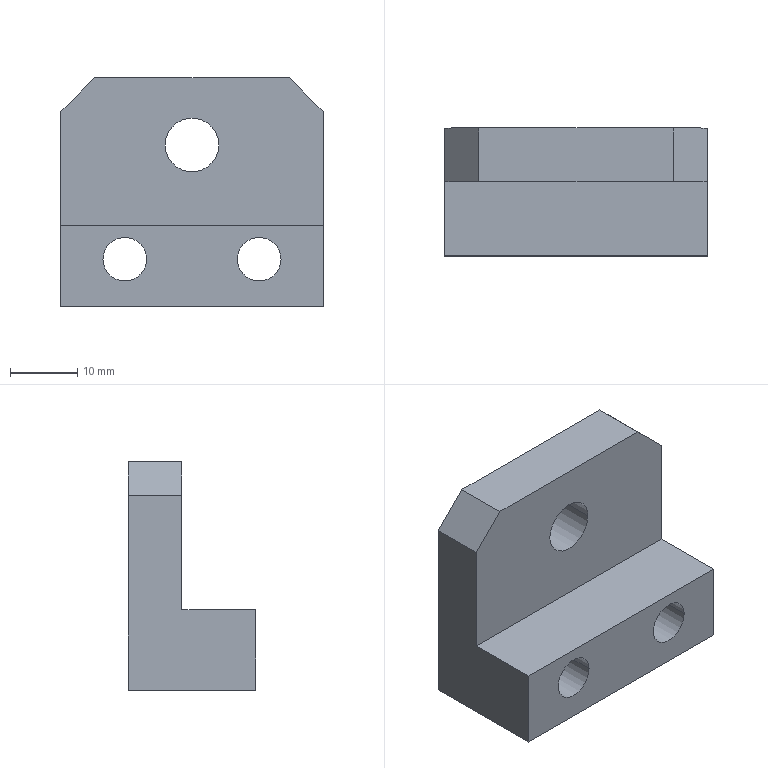Component | SolidWorks | AdjustmentBlock-1 | 1 solid | 22 faces | box 39 x 19 x 34 mm | volume 13089 mm3 | plane 12 | cylinder 10 | commonest cylinder face diameters 11 x4 6.5 x4 8 x2
build123d program:
from build123d import *

# Parameters (mm, degrees)
SKETCH1_W                                          = 39
SKETCH1_H                                          = 34
BOSS_EXTRUDE1_DEPTH                                = 19
SKETCH2_W                                          = 39
SKETCH2_H                                          = 22
CUT_EXTRUDE1_DEPTH                                 = 11
HOLE_SIZE_ACCORDING_TO_TYPE_1_OF_HEXAG_D           = 6.5
HOLE_SIZE_ACCORDING_TO_TYPE_1_OF_HEXAG_CBORE_D     = 11
HOLE_SIZE_ACCORDING_TO_TYPE_1_OF_HEXAG_CBORE_DEPTH = 6.5
SKETCH5_R                                          = 4
CUT_EXTRUDE2_DEPTH                                 = 11
CHAMFER1_SIZE                                      = 5


with BuildPart() as part:
    # Sketch1 → Boss-Extrude1 (new body)
    with BuildSketch(Plane.XY):
        Rectangle(SKETCH1_W, SKETCH1_H)
    extrude(amount=BOSS_EXTRUDE1_DEPTH)

    # Sketch2 → Cut-Extrude1 (cut)
    with BuildSketch(Plane(origin=(0, 0, 0), x_dir=(-1, 0, 0), z_dir=(0, 0, -1))):
        with Locations((0, 6)):
            Rectangle(SKETCH2_W, SKETCH2_H)
    extrude(amount=-CUT_EXTRUDE1_DEPTH, mode=Mode.SUBTRACT)

    # Hole Size _according to_ Type 1 of Hexag (through all)
    with Locations(Plane(origin=(-10, -10, 19), x_dir=(1, 0, 0), z_dir=(0, 0, 1))):
        with Locations((0, 0), (20, 0)):
            CounterBoreHole(HOLE_SIZE_ACCORDING_TO_TYPE_1_OF_HEXAG_D / 2, HOLE_SIZE_ACCORDING_TO_TYPE_1_OF_HEXAG_CBORE_D / 2, HOLE_SIZE_ACCORDING_TO_TYPE_1_OF_HEXAG_CBORE_DEPTH)

    # Sketch5 → Cut-Extrude2 (cut)
    with BuildSketch(Plane.XY.offset(19)):
        with Locations((0, 7)):
            Circle(SKETCH5_R)
    extrude(amount=-CUT_EXTRUDE2_DEPTH, mode=Mode.SUBTRACT)

    # Chamfer1
    chamfer1_edges = [part.edges().sort_by_distance(p)[0] for p in [
        (-19.5, 17, 15),
        (19.5, 17, 15),
    ]]
    chamfer(chamfer1_edges, length=CHAMFER1_SIZE)


solid = part.part

# Placed as in the assembly
solid = solid.moved(Location((-48.047, 25.96, 8), (-90, 0, 180)))
STEP:
#1=COLOUR_RGB('',0.7922,0.8196,0.9333);
#2=FILL_AREA_STYLE_COLOUR('',#1);
#3=FILL_AREA_STYLE('',(#2));
#4=SURFACE_STYLE_FILL_AREA(#3);
#5=SURFACE_SIDE_STYLE('',(#4));
#6=SURFACE_STYLE_USAGE(.BOTH.,#5);
#7=PRESENTATION_STYLE_ASSIGNMENT((#6));
#8=CARTESIAN_POINT('',(-2.049,1.455,0.5906));
#9=VERTEX_POINT('',#8);
#10=CARTESIAN_POINT('',(-1.734,1.455,0.5906));
#11=VERTEX_POINT('',#10);
#12=CARTESIAN_POINT('',(-1.892,1.455,0.5906));
#13=DIRECTION('',(0.,-1.,0.));
#14=DIRECTION('',(1.,0.,0.));
#15=AXIS2_PLACEMENT_3D('',#12,#13,#14);
#16=CIRCLE('',#15,0.1575);
#17=EDGE_CURVE('',#9,#11,#16,.T.);
#18=ORIENTED_EDGE('',*,*,#17,.T.);
#19=CARTESIAN_POINT('',(-1.734,1.77,0.5906));
#20=VERTEX_POINT('',#19);
#21=CARTESIAN_POINT('',(-1.734,1.337,0.5906));
#22=DIRECTION('',(0.,1.,0.));
#23=VECTOR('',#22,39.37);
#24=LINE('',#21,#23);
#25=EDGE_CURVE('',#11,#20,#24,.T.);
#26=ORIENTED_EDGE('',*,*,#25,.T.);
#27=CARTESIAN_POINT('',(-2.049,1.77,0.5906));
#28=VERTEX_POINT('',#27);
#29=CARTESIAN_POINT('',(-1.892,1.77,0.5906));
#30=DIRECTION('',(0.,1.,0.));
#31=DIRECTION('',(-1.,0.,0.));
#32=AXIS2_PLACEMENT_3D('',#29,#30,#31);
#33=CIRCLE('',#32,0.1575);
#34=EDGE_CURVE('',#20,#28,#33,.T.);
#35=ORIENTED_EDGE('',*,*,#34,.T.);
#36=CARTESIAN_POINT('',(-2.049,1.337,0.5906));
#37=DIRECTION('',(0.,1.,0.));
#38=VECTOR('',#37,39.37);
#39=LINE('',#36,#38);
#40=EDGE_CURVE('',#9,#28,#39,.T.);
#41=ORIENTED_EDGE('',*,*,#40,.F.);
#42=EDGE_LOOP('',(#18,#26,#35,#41));
#43=FACE_OUTER_BOUND('',#42,.T.);
#44=CARTESIAN_POINT('',(-1.892,1.337,0.5906));
#45=DIRECTION('',(0.,1.,0.));
#46=DIRECTION('',(-1.,0.,0.));
#47=AXIS2_PLACEMENT_3D('',#44,#45,#46);
#48=CYLINDRICAL_SURFACE('',#47,0.1575);
#49=ADVANCED_FACE('',(#43),#48,.F.);
#50=CARTESIAN_POINT('',(-1.281,1.514,-0.07874));
#51=VERTEX_POINT('',#50);
#52=CARTESIAN_POINT('',(-1.714,1.514,-0.07874));
#53=VERTEX_POINT('',#52);
#54=CARTESIAN_POINT('',(-1.498,1.514,-0.07874));
#55=DIRECTION('',(0.,1.,0.));
#56=DIRECTION('',(-1.,0.,0.));
#57=AXIS2_PLACEMENT_3D('',#54,#55,#56);
#58=CIRCLE('',#57,0.2165);
#59=EDGE_CURVE('',#51,#53,#58,.T.);
#60=ORIENTED_EDGE('',*,*,#59,.F.);
#61=CARTESIAN_POINT('',(-1.281,1.77,-0.07874));
#62=VERTEX_POINT('',#61);
#63=CARTESIAN_POINT('',(-1.281,1.77,-0.07874));
#64=DIRECTION('',(0.,1.,0.));
#65=VECTOR('',#64,39.37);
#66=LINE('',#63,#65);
#67=EDGE_CURVE('',#51,#62,#66,.T.);
#68=ORIENTED_EDGE('',*,*,#67,.T.);
#69=CARTESIAN_POINT('',(-1.714,1.77,-0.07874));
#70=VERTEX_POINT('',#69);
#71=CARTESIAN_POINT('',(-1.498,1.77,-0.07874));
#72=DIRECTION('',(0.,1.,0.));
#73=DIRECTION('',(-1.,0.,0.));
#74=AXIS2_PLACEMENT_3D('',#71,#72,#73);
#75=CIRCLE('',#74,0.2165);
#76=EDGE_CURVE('',#62,#70,#75,.T.);
#77=ORIENTED_EDGE('',*,*,#76,.T.);
#78=CARTESIAN_POINT('',(-1.714,1.77,-0.07874));
#79=DIRECTION('',(0.,1.,0.));
#80=VECTOR('',#79,39.37);
#81=LINE('',#78,#80);
#82=EDGE_CURVE('',#53,#70,#81,.T.);
#83=ORIENTED_EDGE('',*,*,#82,.F.);
#84=EDGE_LOOP('',(#60,#68,#77,#83));
#85=FACE_OUTER_BOUND('',#84,.T.);
#86=CARTESIAN_POINT('',(-1.498,1.77,-0.07874));
#87=DIRECTION('',(0.,1.,0.));
#88=DIRECTION('',(-1.,0.,0.));
#89=AXIS2_PLACEMENT_3D('',#86,#87,#88);
#90=CYLINDRICAL_SURFACE('',#89,0.2165);
#91=ADVANCED_FACE('',(#85),#90,.F.);
#92=CARTESIAN_POINT('',(-1.626,1.022,-0.07874));
#93=VERTEX_POINT('',#92);
#94=CARTESIAN_POINT('',(-1.37,1.022,-0.07874));
#95=VERTEX_POINT('',#94);
#96=CARTESIAN_POINT('',(-1.498,1.022,-0.07874));
#97=DIRECTION('',(0.,-1.,0.));
#98=DIRECTION('',(1.,0.,0.));
#99=AXIS2_PLACEMENT_3D('',#96,#97,#98);
#100=CIRCLE('',#99,0.128);
#101=EDGE_CURVE('',#93,#95,#100,.T.);
#102=ORIENTED_EDGE('',*,*,#101,.T.);
#103=CARTESIAN_POINT('',(-1.37,1.514,-0.07874));
#104=VERTEX_POINT('',#103);
#105=CARTESIAN_POINT('',(-1.37,1.77,-0.07874));
#106=DIRECTION('',(0.,1.,0.));
#107=VECTOR('',#106,39.37);
#108=LINE('',#105,#107);
#109=EDGE_CURVE('',#95,#104,#108,.T.);
#110=ORIENTED_EDGE('',*,*,#109,.T.);
#111=CARTESIAN_POINT('',(-1.626,1.514,-0.07874));
#112=VERTEX_POINT('',#111);
#113=CARTESIAN_POINT('',(-1.498,1.514,-0.07874));
#114=DIRECTION('',(0.,1.,0.));
#115=DIRECTION('',(-1.,0.,0.));
#116=AXIS2_PLACEMENT_3D('',#113,#114,#115);
#117=CIRCLE('',#116,0.128);
#118=EDGE_CURVE('',#104,#112,#117,.T.);
#119=ORIENTED_EDGE('',*,*,#118,.T.);
#120=CARTESIAN_POINT('',(-1.626,1.77,-0.07874));
#121=DIRECTION('',(0.,1.,0.));
#122=VECTOR('',#121,39.37);
#123=LINE('',#120,#122);
#124=EDGE_CURVE('',#93,#112,#123,.T.);
#125=ORIENTED_EDGE('',*,*,#124,.F.);
#126=EDGE_LOOP('',(#102,#110,#119,#125));
#127=FACE_OUTER_BOUND('',#126,.T.);
#128=CARTESIAN_POINT('',(-1.498,1.77,-0.07874));
#129=DIRECTION('',(0.,1.,0.));
#130=DIRECTION('',(-1.,0.,0.));
#131=AXIS2_PLACEMENT_3D('',#128,#129,#130);
#132=CYLINDRICAL_SURFACE('',#131,0.128);
#133=ADVANCED_FACE('',(#127),#132,.F.);
#134=CARTESIAN_POINT('',(-2.069,1.514,-0.07874));
#135=VERTEX_POINT('',#134);
#136=CARTESIAN_POINT('',(-2.502,1.514,-0.07874));
#137=VERTEX_POINT('',#136);
#138=CARTESIAN_POINT('',(-2.285,1.514,-0.07874));
#139=DIRECTION('',(0.,1.,0.));
#140=DIRECTION('',(-1.,0.,0.));
#141=AXIS2_PLACEMENT_3D('',#138,#139,#140);
#142=CIRCLE('',#141,0.2165);
#143=EDGE_CURVE('',#135,#137,#142,.T.);
#144=ORIENTED_EDGE('',*,*,#143,.F.);
#145=CARTESIAN_POINT('',(-2.069,1.77,-0.07874));
#146=VERTEX_POINT('',#145);
#147=CARTESIAN_POINT('',(-2.069,1.77,-0.07874));
#148=DIRECTION('',(0.,1.,0.));
#149=VECTOR('',#148,39.37);
#150=LINE('',#147,#149);
#151=EDGE_CURVE('',#135,#146,#150,.T.);
#152=ORIENTED_EDGE('',*,*,#151,.T.);
#153=CARTESIAN_POINT('',(-2.502,1.77,-0.07874));
#154=VERTEX_POINT('',#153);
#155=CARTESIAN_POINT('',(-2.285,1.77,-0.07874));
#156=DIRECTION('',(0.,1.,0.));
#157=DIRECTION('',(-1.,0.,0.));
#158=AXIS2_PLACEMENT_3D('',#155,#156,#157);
#159=CIRCLE('',#158,0.2165);
#160=EDGE_CURVE('',#146,#154,#159,.T.);
#161=ORIENTED_EDGE('',*,*,#160,.T.);
#162=CARTESIAN_POINT('',(-2.502,1.77,-0.07874));
#163=DIRECTION('',(0.,1.,0.));
#164=VECTOR('',#163,39.37);
#165=LINE('',#162,#164);
#166=EDGE_CURVE('',#137,#154,#165,.T.);
#167=ORIENTED_EDGE('',*,*,#166,.F.);
#168=EDGE_LOOP('',(#144,#152,#161,#167));
#169=FACE_OUTER_BOUND('',#168,.T.);
#170=CARTESIAN_POINT('',(-2.285,1.77,-0.07874));
#171=DIRECTION('',(0.,1.,0.));
#172=DIRECTION('',(-1.,0.,0.));
#173=AXIS2_PLACEMENT_3D('',#170,#171,#172);
#174=CYLINDRICAL_SURFACE('',#173,0.2165);
#175=ADVANCED_FACE('',(#169),#174,.F.);
#176=CARTESIAN_POINT('',(-2.413,1.022,-0.07874));
#177=VERTEX_POINT('',#176);
#178=CARTESIAN_POINT('',(-2.157,1.022,-0.07874));
#179=VERTEX_POINT('',#178);
#180=CARTESIAN_POINT('',(-2.285,1.022,-0.07874));
#181=DIRECTION('',(0.,-1.,0.));
#182=DIRECTION('',(1.,0.,0.));
#183=AXIS2_PLACEMENT_3D('',#180,#181,#182);
#184=CIRCLE('',#183,0.128);
#185=EDGE_CURVE('',#177,#179,#184,.T.);
#186=ORIENTED_EDGE('',*,*,#185,.T.);
#187=CARTESIAN_POINT('',(-2.157,1.514,-0.07874));
#188=VERTEX_POINT('',#187);
#189=CARTESIAN_POINT('',(-2.157,1.77,-0.07874));
#190=DIRECTION('',(0.,1.,0.));
#191=VECTOR('',#190,39.37);
#192=LINE('',#189,#191);
#193=EDGE_CURVE('',#179,#188,#192,.T.);
#194=ORIENTED_EDGE('',*,*,#193,.T.);
#195=CARTESIAN_POINT('',(-2.413,1.514,-0.07874));
#196=VERTEX_POINT('',#195);
#197=CARTESIAN_POINT('',(-2.285,1.514,-0.07874));
#198=DIRECTION('',(0.,1.,0.));
#199=DIRECTION('',(-1.,0.,0.));
#200=AXIS2_PLACEMENT_3D('',#197,#198,#199);
#201=CIRCLE('',#200,0.128);
#202=EDGE_CURVE('',#188,#196,#201,.T.);
#203=ORIENTED_EDGE('',*,*,#202,.T.);
#204=CARTESIAN_POINT('',(-2.413,1.77,-0.07874));
#205=DIRECTION('',(0.,1.,0.));
#206=VECTOR('',#205,39.37);
#207=LINE('',#204,#206);
#208=EDGE_CURVE('',#177,#196,#207,.T.);
#209=ORIENTED_EDGE('',*,*,#208,.F.);
#210=EDGE_LOOP('',(#186,#194,#203,#209));
#211=FACE_OUTER_BOUND('',#210,.T.);
#212=CARTESIAN_POINT('',(-2.285,1.77,-0.07874));
#213=DIRECTION('',(0.,1.,0.));
#214=DIRECTION('',(-1.,0.,0.));
#215=AXIS2_PLACEMENT_3D('',#212,#213,#214);
#216=CYLINDRICAL_SURFACE('',#215,0.128);
#217=ADVANCED_FACE('',(#211),#216,.F.);
#218=CARTESIAN_POINT('',(-2.462,1.77,0.9843));
#219=VERTEX_POINT('',#218);
#220=CARTESIAN_POINT('',(-1.321,1.77,0.9843));
#221=VERTEX_POINT('',#220);
#222=CARTESIAN_POINT('',(-1.124,1.77,0.9843));
#223=DIRECTION('',(1.,0.,0.));
#224=VECTOR('',#223,39.37);
#225=LINE('',#222,#224);
#226=EDGE_CURVE('',#219,#221,#225,.T.);
#227=ORIENTED_EDGE('',*,*,#226,.F.);
#228=CARTESIAN_POINT('',(-2.462,1.455,0.9843));
#229=VERTEX_POINT('',#228);
#230=CARTESIAN_POINT('',(-2.462,1.77,0.9843));
#231=DIRECTION('',(0.,-1.,0.));
#232=VECTOR('',#231,39.37);
#233=LINE('',#230,#232);
#234=EDGE_CURVE('',#219,#229,#233,.T.);
#235=ORIENTED_EDGE('',*,*,#234,.T.);
#236=CARTESIAN_POINT('',(-1.321,1.455,0.9843));
#237=VERTEX_POINT('',#236);
#238=CARTESIAN_POINT('',(-2.659,1.455,0.9843));
#239=DIRECTION('',(-1.,0.,0.));
#240=VECTOR('',#239,39.37);
#241=LINE('',#238,#240);
#242=EDGE_CURVE('',#237,#229,#241,.T.);
#243=ORIENTED_EDGE('',*,*,#242,.F.);
#244=CARTESIAN_POINT('',(-1.321,1.77,0.9843));
#245=DIRECTION('',(0.,1.,0.));
#246=VECTOR('',#245,39.37);
#247=LINE('',#244,#246);
#248=EDGE_CURVE('',#237,#221,#247,.T.);
#249=ORIENTED_EDGE('',*,*,#248,.T.);
#250=EDGE_LOOP('',(#227,#235,#243,#249));
#251=FACE_OUTER_BOUND('',#250,.T.);
#252=CARTESIAN_POINT('',(-1.124,1.77,0.9843));
#253=DIRECTION('',(0.,0.,-1.));
#254=DIRECTION('',(0.,-1.,0.));
#255=AXIS2_PLACEMENT_3D('',#252,#253,#254);
#256=PLANE('',#255);
#257=ADVANCED_FACE('',(#251),#256,.F.);
#258=CARTESIAN_POINT('',(-2.659,1.455,0.7874));
#259=VERTEX_POINT('',#258);
#260=CARTESIAN_POINT('',(-2.659,1.455,0.1181));
#261=VERTEX_POINT('',#260);
#262=CARTESIAN_POINT('',(-2.659,1.455,0.9843));
#263=DIRECTION('',(0.,0.,-1.));
#264=VECTOR('',#263,39.37);
#265=LINE('',#262,#264);
#266=EDGE_CURVE('',#259,#261,#265,.T.);
#267=ORIENTED_EDGE('',*,*,#266,.F.);
#268=CARTESIAN_POINT('',(-2.659,1.77,0.7874));
#269=VERTEX_POINT('',#268);
#270=CARTESIAN_POINT('',(-2.659,1.77,0.7874));
#271=DIRECTION('',(0.,1.,0.));
#272=VECTOR('',#271,39.37);
#273=LINE('',#270,#272);
#274=EDGE_CURVE('',#259,#269,#273,.T.);
#275=ORIENTED_EDGE('',*,*,#274,.T.);
#276=CARTESIAN_POINT('',(-2.659,1.77,-0.3543));
#277=VERTEX_POINT('',#276);
#278=CARTESIAN_POINT('',(-2.659,1.77,-0.3543));
#279=DIRECTION('',(0.,0.,1.));
#280=VECTOR('',#279,39.37);
#281=LINE('',#278,#280);
#282=EDGE_CURVE('',#277,#269,#281,.T.);
#283=ORIENTED_EDGE('',*,*,#282,.F.);
#284=CARTESIAN_POINT('',(-2.659,1.022,-0.3543));
#285=VERTEX_POINT('',#284);
#286=CARTESIAN_POINT('',(-2.659,1.77,-0.3543));
#287=DIRECTION('',(0.,-1.,0.));
#288=VECTOR('',#287,39.37);
#289=LINE('',#286,#288);
#290=EDGE_CURVE('',#277,#285,#289,.T.);
#291=ORIENTED_EDGE('',*,*,#290,.T.);
#292=CARTESIAN_POINT('',(-2.659,1.022,0.1181));
#293=VERTEX_POINT('',#292);
#294=CARTESIAN_POINT('',(-2.659,1.022,-0.3543));
#295=DIRECTION('',(0.,0.,1.));
#296=VECTOR('',#295,39.37);
#297=LINE('',#294,#296);
#298=EDGE_CURVE('',#285,#293,#297,.T.);
#299=ORIENTED_EDGE('',*,*,#298,.T.);
#300=CARTESIAN_POINT('',(-2.659,1.455,0.1181));
#301=DIRECTION('',(0.,-1.,0.));
#302=VECTOR('',#301,39.37);
#303=LINE('',#300,#302);
#304=EDGE_CURVE('',#261,#293,#303,.T.);
#305=ORIENTED_EDGE('',*,*,#304,.F.);
#306=EDGE_LOOP('',(#267,#275,#283,#291,#299,#305));
#307=FACE_OUTER_BOUND('',#306,.T.);
#308=CARTESIAN_POINT('',(-2.659,1.77,-0.3543));
#309=DIRECTION('',(1.,0.,0.));
#310=DIRECTION('',(0.,1.,0.));
#311=AXIS2_PLACEMENT_3D('',#308,#309,#310);
#312=PLANE('',#311);
#313=ADVANCED_FACE('',(#307),#312,.F.);
#314=CARTESIAN_POINT('',(-1.124,1.77,0.7874));
#315=VERTEX_POINT('',#314);
#316=CARTESIAN_POINT('',(-1.124,1.77,-0.3543));
#317=VERTEX_POINT('',#316);
#318=CARTESIAN_POINT('',(-1.124,1.77,-0.3543));
#319=DIRECTION('',(0.,0.,-1.));
#320=VECTOR('',#319,39.37);
#321=LINE('',#318,#320);
#322=EDGE_CURVE('',#315,#317,#321,.T.);
#323=ORIENTED_EDGE('',*,*,#322,.F.);
#324=CARTESIAN_POINT('',(-1.124,1.455,0.7874));
#325=VERTEX_POINT('',#324);
#326=CARTESIAN_POINT('',(-1.124,1.77,0.7874));
#327=DIRECTION('',(0.,-1.,0.));
#328=VECTOR('',#327,39.37);
#329=LINE('',#326,#328);
#330=EDGE_CURVE('',#315,#325,#329,.T.);
#331=ORIENTED_EDGE('',*,*,#330,.T.);
#332=CARTESIAN_POINT('',(-1.124,1.455,0.1181));
#333=VERTEX_POINT('',#332);
#334=CARTESIAN_POINT('',(-1.124,1.455,0.9843));
#335=DIRECTION('',(0.,0.,1.));
#336=VECTOR('',#335,39.37);
#337=LINE('',#334,#336);
#338=EDGE_CURVE('',#333,#325,#337,.T.);
#339=ORIENTED_EDGE('',*,*,#338,.F.);
#340=CARTESIAN_POINT('',(-1.124,1.022,0.1181));
#341=VERTEX_POINT('',#340);
#342=CARTESIAN_POINT('',(-1.124,1.455,0.1181));
#343=DIRECTION('',(0.,-1.,0.));
#344=VECTOR('',#343,39.37);
#345=LINE('',#342,#344);
#346=EDGE_CURVE('',#333,#341,#345,.T.);
#347=ORIENTED_EDGE('',*,*,#346,.T.);
#348=CARTESIAN_POINT('',(-1.124,1.022,-0.3543));
#349=VERTEX_POINT('',#348);
#350=CARTESIAN_POINT('',(-1.124,1.022,-0.3543));
#351=DIRECTION('',(0.,0.,-1.));
#352=VECTOR('',#351,39.37);
#353=LINE('',#350,#352);
#354=EDGE_CURVE('',#341,#349,#353,.T.);
#355=ORIENTED_EDGE('',*,*,#354,.T.);
#356=CARTESIAN_POINT('',(-1.124,1.77,-0.3543));
#357=DIRECTION('',(0.,-1.,0.));
#358=VECTOR('',#357,39.37);
#359=LINE('',#356,#358);
#360=EDGE_CURVE('',#317,#349,#359,.T.);
#361=ORIENTED_EDGE('',*,*,#360,.F.);
#362=EDGE_LOOP('',(#323,#331,#339,#347,#355,#361));
#363=FACE_OUTER_BOUND('',#362,.T.);
#364=CARTESIAN_POINT('',(-1.124,1.77,-0.3543));
#365=DIRECTION('',(-1.,0.,0.));
#366=DIRECTION('',(0.,-1.,0.));
#367=AXIS2_PLACEMENT_3D('',#364,#365,#366);
#368=PLANE('',#367);
#369=ADVANCED_FACE('',(#363),#368,.F.);
#370=CARTESIAN_POINT('',(-1.124,1.022,-0.3543));
#371=DIRECTION('',(-1.,0.,0.));
#372=VECTOR('',#371,39.37);
#373=LINE('',#370,#372);
#374=EDGE_CURVE('',#349,#285,#373,.T.);
#375=ORIENTED_EDGE('',*,*,#374,.T.);
#376=ORIENTED_EDGE('',*,*,#290,.F.);
#377=CARTESIAN_POINT('',(-1.124,1.77,-0.3543));
#378=DIRECTION('',(-1.,0.,0.));
#379=VECTOR('',#378,39.37);
#380=LINE('',#377,#379);
#381=EDGE_CURVE('',#317,#277,#380,.T.);
#382=ORIENTED_EDGE('',*,*,#381,.F.);
#383=ORIENTED_EDGE('',*,*,#360,.T.);
#384=EDGE_LOOP('',(#375,#376,#382,#383));
#385=FACE_OUTER_BOUND('',#384,.T.);
#386=CARTESIAN_POINT('',(-1.124,1.77,-0.3543));
#387=DIRECTION('',(0.,0.,1.));
#388=DIRECTION('',(0.,1.,0.));
#389=AXIS2_PLACEMENT_3D('',#386,#387,#388);
#390=PLANE('',#389);
#391=ADVANCED_FACE('',(#385),#390,.F.);
#392=CARTESIAN_POINT('',(-1.892,1.77,0.5906));
#393=DIRECTION('',(0.,1.,0.));
#394=DIRECTION('',(-1.,0.,0.));
#395=AXIS2_PLACEMENT_3D('',#392,#393,#394);
#396=CIRCLE('',#395,0.1575);
#397=EDGE_CURVE('',#28,#20,#396,.T.);
#398=ORIENTED_EDGE('',*,*,#397,.F.);
#399=ORIENTED_EDGE('',*,*,#34,.F.);
#400=EDGE_LOOP('',(#398,#399));
#401=FACE_BOUND('',#400,.T.);
#402=CARTESIAN_POINT('',(-1.498,1.77,-0.07874));
#403=DIRECTION('',(0.,1.,0.));
#404=DIRECTION('',(-1.,0.,0.));
#405=AXIS2_PLACEMENT_3D('',#402,#403,#404);
#406=CIRCLE('',#405,0.2165);
#407=EDGE_CURVE('',#70,#62,#406,.T.);
#408=ORIENTED_EDGE('',*,*,#407,.F.);
#409=ORIENTED_EDGE('',*,*,#76,.F.);
#410=EDGE_LOOP('',(#408,#409));
#411=FACE_BOUND('',#410,.T.);
#412=CARTESIAN_POINT('',(-2.285,1.77,-0.07874));
#413=DIRECTION('',(0.,1.,0.));
#414=DIRECTION('',(-1.,0.,0.));
#415=AXIS2_PLACEMENT_3D('',#412,#413,#414);
#416=CIRCLE('',#415,0.2165);
#417=EDGE_CURVE('',#154,#146,#416,.T.);
#418=ORIENTED_EDGE('',*,*,#417,.F.);
#419=ORIENTED_EDGE('',*,*,#160,.F.);
#420=EDGE_LOOP('',(#418,#419));
#421=FACE_BOUND('',#420,.T.);
#422=ORIENTED_EDGE('',*,*,#282,.T.);
#423=CARTESIAN_POINT('',(-2.462,1.77,0.9843));
#424=DIRECTION('',(0.7071,0.,0.7071));
#425=VECTOR('',#424,39.37);
#426=LINE('',#423,#425);
#427=EDGE_CURVE('',#269,#219,#426,.T.);
#428=ORIENTED_EDGE('',*,*,#427,.T.);
#429=ORIENTED_EDGE('',*,*,#226,.T.);
#430=CARTESIAN_POINT('',(-1.124,1.77,0.7874));
#431=DIRECTION('',(0.7071,0.,-0.7071));
#432=VECTOR('',#431,39.37);
#433=LINE('',#430,#432);
#434=EDGE_CURVE('',#221,#315,#433,.T.);
#435=ORIENTED_EDGE('',*,*,#434,.T.);
#436=ORIENTED_EDGE('',*,*,#322,.T.);
#437=ORIENTED_EDGE('',*,*,#381,.T.);
#438=EDGE_LOOP('',(#422,#428,#429,#435,#436,#437));
#439=FACE_OUTER_BOUND('',#438,.T.);
#440=CARTESIAN_POINT('',(-1.892,1.77,0.315));
#441=DIRECTION('',(0.,-1.,0.));
#442=DIRECTION('',(1.,0.,0.));
#443=AXIS2_PLACEMENT_3D('',#440,#441,#442);
#444=PLANE('',#443);
#445=ADVANCED_FACE('',(#401,#411,#421,#439),#444,.F.);
#446=ORIENTED_EDGE('',*,*,#101,.F.);
#447=CARTESIAN_POINT('',(-1.498,1.022,-0.07874));
#448=DIRECTION('',(0.,-1.,0.));
#449=DIRECTION('',(1.,0.,0.));
#450=AXIS2_PLACEMENT_3D('',#447,#448,#449);
#451=CIRCLE('',#450,0.128);
#452=EDGE_CURVE('',#95,#93,#451,.T.);
#453=ORIENTED_EDGE('',*,*,#452,.F.);
#454=EDGE_LOOP('',(#446,#453));
#455=FACE_BOUND('',#454,.T.);
#456=ORIENTED_EDGE('',*,*,#185,.F.);
#457=CARTESIAN_POINT('',(-2.285,1.022,-0.07874));
#458=DIRECTION('',(0.,-1.,0.));
#459=DIRECTION('',(1.,0.,0.));
#460=AXIS2_PLACEMENT_3D('',#457,#458,#459);
#461=CIRCLE('',#460,0.128);
#462=EDGE_CURVE('',#179,#177,#461,.T.);
#463=ORIENTED_EDGE('',*,*,#462,.F.);
#464=EDGE_LOOP('',(#456,#463));
#465=FACE_BOUND('',#464,.T.);
#466=CARTESIAN_POINT('',(-2.659,1.022,0.1181));
#467=DIRECTION('',(1.,0.,0.));
#468=VECTOR('',#467,39.37);
#469=LINE('',#466,#468);
#470=EDGE_CURVE('',#293,#341,#469,.T.);
#471=ORIENTED_EDGE('',*,*,#470,.F.);
#472=ORIENTED_EDGE('',*,*,#298,.F.);
#473=ORIENTED_EDGE('',*,*,#374,.F.);
#474=ORIENTED_EDGE('',*,*,#354,.F.);
#475=EDGE_LOOP('',(#471,#472,#473,#474));
#476=FACE_OUTER_BOUND('',#475,.T.);
#477=CARTESIAN_POINT('',(-1.892,1.022,0.315));
#478=DIRECTION('',(0.,-1.,0.));
#479=DIRECTION('',(1.,0.,0.));
#480=AXIS2_PLACEMENT_3D('',#477,#478,#479);
#481=PLANE('',#480);
#482=ADVANCED_FACE('',(#455,#465,#476),#481,.T.);
#483=ORIENTED_EDGE('',*,*,#470,.T.);
#484=ORIENTED_EDGE('',*,*,#346,.F.);
#485=CARTESIAN_POINT('',(-2.659,1.455,0.1181));
#486=DIRECTION('',(1.,0.,0.));
#487=VECTOR('',#486,39.37);
#488=LINE('',#485,#487);
#489=EDGE_CURVE('',#261,#333,#488,.T.);
#490=ORIENTED_EDGE('',*,*,#489,.F.);
#491=ORIENTED_EDGE('',*,*,#304,.T.);
#492=EDGE_LOOP('',(#483,#484,#490,#491));
#493=FACE_OUTER_BOUND('',#492,.T.);
#494=CARTESIAN_POINT('',(-2.659,1.455,0.1181));
#495=DIRECTION('',(0.,0.,-1.));
#496=DIRECTION('',(0.,-1.,0.));
#497=AXIS2_PLACEMENT_3D('',#494,#495,#496);
#498=PLANE('',#497);
#499=ADVANCED_FACE('',(#493),#498,.F.);
#500=ORIENTED_EDGE('',*,*,#17,.F.);
#501=CARTESIAN_POINT('',(-1.892,1.455,0.5906));
#502=DIRECTION('',(0.,-1.,0.));
#503=DIRECTION('',(1.,0.,0.));
#504=AXIS2_PLACEMENT_3D('',#501,#502,#503);
#505=CIRCLE('',#504,0.1575);
#506=EDGE_CURVE('',#11,#9,#505,.T.);
#507=ORIENTED_EDGE('',*,*,#506,.F.);
#508=EDGE_LOOP('',(#500,#507));
#509=FACE_BOUND('',#508,.T.);
#510=ORIENTED_EDGE('',*,*,#242,.T.);
#511=CARTESIAN_POINT('',(-2.512,1.455,0.935));
#512=DIRECTION('',(-0.7071,0.,-0.7071));
#513=VECTOR('',#512,39.37);
#514=LINE('',#511,#513);
#515=EDGE_CURVE('',#229,#259,#514,.T.);
#516=ORIENTED_EDGE('',*,*,#515,.T.);
#517=ORIENTED_EDGE('',*,*,#266,.T.);
#518=ORIENTED_EDGE('',*,*,#489,.T.);
#519=ORIENTED_EDGE('',*,*,#338,.T.);
#520=CARTESIAN_POINT('',(-1.272,1.455,0.935));
#521=DIRECTION('',(-0.7071,0.,0.7071));
#522=VECTOR('',#521,39.37);
#523=LINE('',#520,#522);
#524=EDGE_CURVE('',#325,#237,#523,.T.);
#525=ORIENTED_EDGE('',*,*,#524,.T.);
#526=EDGE_LOOP('',(#510,#516,#517,#518,#519,#525));
#527=FACE_OUTER_BOUND('',#526,.T.);
#528=CARTESIAN_POINT('',(-1.892,1.455,0.315));
#529=DIRECTION('',(0.,-1.,0.));
#530=DIRECTION('',(1.,0.,0.));
#531=AXIS2_PLACEMENT_3D('',#528,#529,#530);
#532=PLANE('',#531);
#533=ADVANCED_FACE('',(#509,#527),#532,.T.);
#534=ORIENTED_EDGE('',*,*,#193,.F.);
#535=ORIENTED_EDGE('',*,*,#462,.T.);
#536=ORIENTED_EDGE('',*,*,#208,.T.);
#537=CARTESIAN_POINT('',(-2.285,1.514,-0.07874));
#538=DIRECTION('',(0.,1.,0.));
#539=DIRECTION('',(-1.,0.,0.));
#540=AXIS2_PLACEMENT_3D('',#537,#538,#539);
#541=CIRCLE('',#540,0.128);
#542=EDGE_CURVE('',#196,#188,#541,.T.);
#543=ORIENTED_EDGE('',*,*,#542,.T.);
#544=EDGE_LOOP('',(#534,#535,#536,#543));
#545=FACE_OUTER_BOUND('',#544,.T.);
#546=CARTESIAN_POINT('',(-2.285,1.77,-0.07874));
#547=DIRECTION('',(0.,1.,0.));
#548=DIRECTION('',(-1.,0.,0.));
#549=AXIS2_PLACEMENT_3D('',#546,#547,#548);
#550=CYLINDRICAL_SURFACE('',#549,0.128);
#551=ADVANCED_FACE('',(#545),#550,.F.);
#552=ORIENTED_EDGE('',*,*,#542,.F.);
#553=ORIENTED_EDGE('',*,*,#202,.F.);
#554=EDGE_LOOP('',(#552,#553));
#555=FACE_BOUND('',#554,.T.);
#556=CARTESIAN_POINT('',(-2.285,1.514,-0.07874));
#557=DIRECTION('',(0.,1.,0.));
#558=DIRECTION('',(-1.,0.,0.));
#559=AXIS2_PLACEMENT_3D('',#556,#557,#558);
#560=CIRCLE('',#559,0.2165);
#561=EDGE_CURVE('',#137,#135,#560,.T.);
#562=ORIENTED_EDGE('',*,*,#561,.T.);
#563=ORIENTED_EDGE('',*,*,#143,.T.);
#564=EDGE_LOOP('',(#562,#563));
#565=FACE_OUTER_BOUND('',#564,.T.);
#566=CARTESIAN_POINT('',(-2.413,1.514,-0.07874));
#567=DIRECTION('',(0.,-1.,0.));
#568=DIRECTION('',(1.,0.,0.));
#569=AXIS2_PLACEMENT_3D('',#566,#567,#568);
#570=PLANE('',#569);
#571=ADVANCED_FACE('',(#555,#565),#570,.F.);
#572=ORIENTED_EDGE('',*,*,#151,.F.);
#573=ORIENTED_EDGE('',*,*,#561,.F.);
#574=ORIENTED_EDGE('',*,*,#166,.T.);
#575=ORIENTED_EDGE('',*,*,#417,.T.);
#576=EDGE_LOOP('',(#572,#573,#574,#575));
#577=FACE_OUTER_BOUND('',#576,.T.);
#578=CARTESIAN_POINT('',(-2.285,1.77,-0.07874));
#579=DIRECTION('',(0.,1.,0.));
#580=DIRECTION('',(-1.,0.,0.));
#581=AXIS2_PLACEMENT_3D('',#578,#579,#580);
#582=CYLINDRICAL_SURFACE('',#581,0.2165);
#583=ADVANCED_FACE('',(#577),#582,.F.);
#584=ORIENTED_EDGE('',*,*,#109,.F.);
#585=ORIENTED_EDGE('',*,*,#452,.T.);
#586=ORIENTED_EDGE('',*,*,#124,.T.);
#587=CARTESIAN_POINT('',(-1.498,1.514,-0.07874));
#588=DIRECTION('',(0.,1.,0.));
#589=DIRECTION('',(-1.,0.,0.));
#590=AXIS2_PLACEMENT_3D('',#587,#588,#589);
#591=CIRCLE('',#590,0.128);
#592=EDGE_CURVE('',#112,#104,#591,.T.);
#593=ORIENTED_EDGE('',*,*,#592,.T.);
#594=EDGE_LOOP('',(#584,#585,#586,#593));
#595=FACE_OUTER_BOUND('',#594,.T.);
#596=CARTESIAN_POINT('',(-1.498,1.77,-0.07874));
#597=DIRECTION('',(0.,1.,0.));
#598=DIRECTION('',(-1.,0.,0.));
#599=AXIS2_PLACEMENT_3D('',#596,#597,#598);
#600=CYLINDRICAL_SURFACE('',#599,0.128);
#601=ADVANCED_FACE('',(#595),#600,.F.);
#602=ORIENTED_EDGE('',*,*,#592,.F.);
#603=ORIENTED_EDGE('',*,*,#118,.F.);
#604=EDGE_LOOP('',(#602,#603));
#605=FACE_BOUND('',#604,.T.);
#606=CARTESIAN_POINT('',(-1.498,1.514,-0.07874));
#607=DIRECTION('',(0.,1.,0.));
#608=DIRECTION('',(-1.,0.,0.));
#609=AXIS2_PLACEMENT_3D('',#606,#607,#608);
#610=CIRCLE('',#609,0.2165);
#611=EDGE_CURVE('',#53,#51,#610,.T.);
#612=ORIENTED_EDGE('',*,*,#611,.T.);
#613=ORIENTED_EDGE('',*,*,#59,.T.);
#614=EDGE_LOOP('',(#612,#613));
#615=FACE_OUTER_BOUND('',#614,.T.);
#616=CARTESIAN_POINT('',(-1.626,1.514,-0.07874));
#617=DIRECTION('',(0.,-1.,0.));
#618=DIRECTION('',(1.,0.,0.));
#619=AXIS2_PLACEMENT_3D('',#616,#617,#618);
#620=PLANE('',#619);
#621=ADVANCED_FACE('',(#605,#615),#620,.F.);
#622=ORIENTED_EDGE('',*,*,#67,.F.);
#623=ORIENTED_EDGE('',*,*,#611,.F.);
#624=ORIENTED_EDGE('',*,*,#82,.T.);
#625=ORIENTED_EDGE('',*,*,#407,.T.);
#626=EDGE_LOOP('',(#622,#623,#624,#625));
#627=FACE_OUTER_BOUND('',#626,.T.);
#628=CARTESIAN_POINT('',(-1.498,1.77,-0.07874));
#629=DIRECTION('',(0.,1.,0.));
#630=DIRECTION('',(-1.,0.,0.));
#631=AXIS2_PLACEMENT_3D('',#628,#629,#630);
#632=CYLINDRICAL_SURFACE('',#631,0.2165);
#633=ADVANCED_FACE('',(#627),#632,.F.);
#634=ORIENTED_EDGE('',*,*,#25,.F.);
#635=ORIENTED_EDGE('',*,*,#506,.T.);
#636=ORIENTED_EDGE('',*,*,#40,.T.);
#637=ORIENTED_EDGE('',*,*,#397,.T.);
#638=EDGE_LOOP('',(#634,#635,#636,#637));
#639=FACE_OUTER_BOUND('',#638,.T.);
#640=CARTESIAN_POINT('',(-1.892,1.337,0.5906));
#641=DIRECTION('',(0.,1.,0.));
#642=DIRECTION('',(-1.,0.,0.));
#643=AXIS2_PLACEMENT_3D('',#640,#641,#642);
#644=CYLINDRICAL_SURFACE('',#643,0.1575);
#645=ADVANCED_FACE('',(#639),#644,.F.);
#646=ORIENTED_EDGE('',*,*,#427,.F.);
#647=ORIENTED_EDGE('',*,*,#274,.F.);
#648=ORIENTED_EDGE('',*,*,#515,.F.);
#649=ORIENTED_EDGE('',*,*,#234,.F.);
#650=EDGE_LOOP('',(#646,#647,#648,#649));
#651=FACE_OUTER_BOUND('',#650,.T.);
#652=CARTESIAN_POINT('',(-2.462,1.77,0.9843));
#653=DIRECTION('',(0.7071,0.,-0.7071));
#654=DIRECTION('',(0.,-1.,0.));
#655=AXIS2_PLACEMENT_3D('',#652,#653,#654);
#656=PLANE('',#655);
#657=ADVANCED_FACE('',(#651),#656,.F.);
#658=ORIENTED_EDGE('',*,*,#434,.F.);
#659=ORIENTED_EDGE('',*,*,#248,.F.);
#660=ORIENTED_EDGE('',*,*,#524,.F.);
#661=ORIENTED_EDGE('',*,*,#330,.F.);
#662=EDGE_LOOP('',(#658,#659,#660,#661));
#663=FACE_OUTER_BOUND('',#662,.T.);
#664=CARTESIAN_POINT('',(-1.124,1.77,0.7874));
#665=DIRECTION('',(-0.7071,0.,-0.7071));
#666=DIRECTION('',(0.,-1.,0.));
#667=AXIS2_PLACEMENT_3D('',#664,#665,#666);
#668=PLANE('',#667);
#669=ADVANCED_FACE('',(#663),#668,.F.);
#670=CLOSED_SHELL('',(#49,#91,#133,#175,#217,#257,#313,#369,#391,#445,#482,#499,#533,#551,#571,#583,#601,#621,#633,#645,#657,#669));
#671=MANIFOLD_SOLID_BREP('',#670);
#672=STYLED_ITEM('',(#7),#671);
#673=(LENGTH_UNIT()NAMED_UNIT(*)SI_UNIT($,.METRE.));
#674=LENGTH_MEASURE_WITH_UNIT(LENGTH_MEASURE(0.0254),#673);
#675=DIMENSIONAL_EXPONENTS(1.,0.,0.,0.,0.,0.,0.);
#676=(CONVERSION_BASED_UNIT('',#674)LENGTH_UNIT()NAMED_UNIT(#675));
#677=UNCERTAINTY_MEASURE_WITH_UNIT(LENGTH_MEASURE(0.00001),#676,'','');
#678=(NAMED_UNIT(*)PLANE_ANGLE_UNIT()SI_UNIT($,.RADIAN.));
#679=(NAMED_UNIT(*)SI_UNIT($,.STERADIAN.)SOLID_ANGLE_UNIT());
#680=(GEOMETRIC_REPRESENTATION_CONTEXT(3)GLOBAL_UNCERTAINTY_ASSIGNED_CONTEXT((#677))GLOBAL_UNIT_ASSIGNED_CONTEXT((#676,#678,#679))REPRESENTATION_CONTEXT('',''));
#681=MECHANICAL_DESIGN_GEOMETRIC_PRESENTATION_REPRESENTATION('',(#672),#680);
#682=PRESENTATION_LAYER_ASSIGNMENT('','',(#672));
#683=CARTESIAN_POINT('',(0.,0.,0.));
#684=DIRECTION('',(0.,0.,1.));
#685=DIRECTION('',(1.,0.,0.));
#686=AXIS2_PLACEMENT_3D('',#683,#684,#685);
#687=(LENGTH_UNIT()NAMED_UNIT(*)SI_UNIT($,.METRE.));
#688=LENGTH_MEASURE_WITH_UNIT(LENGTH_MEASURE(0.0254),#687);
#689=DIMENSIONAL_EXPONENTS(1.,0.,0.,0.,0.,0.,0.);
#690=(CONVERSION_BASED_UNIT('',#688)LENGTH_UNIT()NAMED_UNIT(#689));
#691=UNCERTAINTY_MEASURE_WITH_UNIT(LENGTH_MEASURE(0.00001),#690,'','');
#692=(NAMED_UNIT(*)PLANE_ANGLE_UNIT()SI_UNIT($,.RADIAN.));
#693=(NAMED_UNIT(*)SI_UNIT($,.STERADIAN.)SOLID_ANGLE_UNIT());
#694=(GEOMETRIC_REPRESENTATION_CONTEXT(3)GLOBAL_UNCERTAINTY_ASSIGNED_CONTEXT((#691))GLOBAL_UNIT_ASSIGNED_CONTEXT((#690,#692,#693))REPRESENTATION_CONTEXT('',''));
#695=ADVANCED_BREP_SHAPE_REPRESENTATION('',(#671,#686),#694);